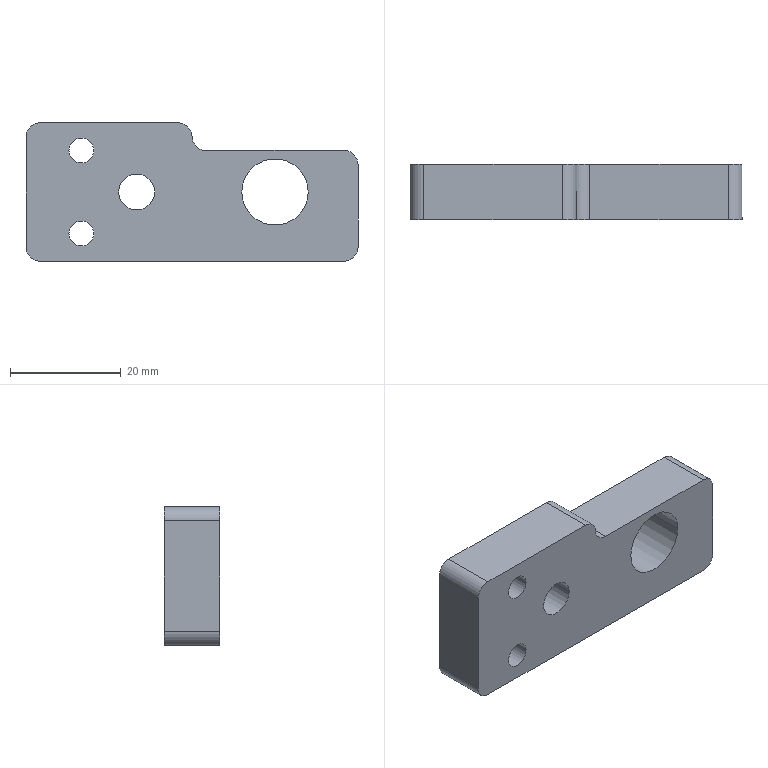Component | SolidWorks | GbgbGuidePlate120F8-1 | 1 solid | 27 faces | box 60 x 10 x 25 mm | volume 11349 mm3 | cylinder 18 | plane 9 | commonest cylinder face diameters 5 x6 8 x4 4.5 x4 12 x2 6.5 x2
STEP:
#1=COLOUR_RGB('',0.7922,0.8196,0.9333);
#2=FILL_AREA_STYLE_COLOUR('',#1);
#3=FILL_AREA_STYLE('',(#2));
#4=SURFACE_STYLE_FILL_AREA(#3);
#5=SURFACE_SIDE_STYLE('',(#4));
#6=SURFACE_STYLE_USAGE(.BOTH.,#5);
#7=PRESENTATION_STYLE_ASSIGNMENT((#6));
#8=CARTESIAN_POINT('',(1.632,15.466,17.234));
#9=VERTEX_POINT('',#8);
#10=CARTESIAN_POINT('',(1.947,15.466,17.234));
#11=VERTEX_POINT('',#10);
#12=CARTESIAN_POINT('',(1.789,15.466,17.234));
#13=DIRECTION('',(-0.,1.,0.));
#14=DIRECTION('',(1.,0.,0.));
#15=AXIS2_PLACEMENT_3D('',#12,#13,#14);
#16=CIRCLE('',#15,0.1575);
#17=EDGE_CURVE('',#9,#11,#16,.T.);
#18=ORIENTED_EDGE('',*,*,#17,.F.);
#19=CARTESIAN_POINT('',(1.632,15.647,17.234));
#20=VERTEX_POINT('',#19);
#21=CARTESIAN_POINT('',(1.632,15.647,17.234));
#22=DIRECTION('',(-0.,1.,0.));
#23=VECTOR('',#22,39.37);
#24=LINE('',#21,#23);
#25=EDGE_CURVE('',#9,#20,#24,.T.);
#26=ORIENTED_EDGE('',*,*,#25,.T.);
#27=CARTESIAN_POINT('',(1.947,15.647,17.234));
#28=VERTEX_POINT('',#27);
#29=CARTESIAN_POINT('',(1.789,15.647,17.234));
#30=DIRECTION('',(-0.,1.,0.));
#31=DIRECTION('',(1.,0.,0.));
#32=AXIS2_PLACEMENT_3D('',#29,#30,#31);
#33=CIRCLE('',#32,0.1575);
#34=EDGE_CURVE('',#20,#28,#33,.T.);
#35=ORIENTED_EDGE('',*,*,#34,.T.);
#36=CARTESIAN_POINT('',(1.947,15.647,17.234));
#37=DIRECTION('',(-0.,1.,0.));
#38=VECTOR('',#37,39.37);
#39=LINE('',#36,#38);
#40=EDGE_CURVE('',#11,#28,#39,.T.);
#41=ORIENTED_EDGE('',*,*,#40,.F.);
#42=EDGE_LOOP('',(#18,#26,#35,#41));
#43=FACE_OUTER_BOUND('',#42,.T.);
#44=CARTESIAN_POINT('',(1.789,15.647,17.234));
#45=DIRECTION('',(-0.,1.,0.));
#46=DIRECTION('',(1.,0.,0.));
#47=AXIS2_PLACEMENT_3D('',#44,#45,#46);
#48=CYLINDRICAL_SURFACE('',#47,0.1575);
#49=ADVANCED_FACE('',(#43),#48,.F.);
#50=CARTESIAN_POINT('',(1.701,15.254,17.234));
#51=VERTEX_POINT('',#50);
#52=CARTESIAN_POINT('',(1.878,15.254,17.234));
#53=VERTEX_POINT('',#52);
#54=CARTESIAN_POINT('',(1.789,15.254,17.234));
#55=DIRECTION('',(-0.,1.,0.));
#56=DIRECTION('',(1.,0.,0.));
#57=AXIS2_PLACEMENT_3D('',#54,#55,#56);
#58=CIRCLE('',#57,0.08858);
#59=EDGE_CURVE('',#51,#53,#58,.T.);
#60=ORIENTED_EDGE('',*,*,#59,.F.);
#61=CARTESIAN_POINT('',(1.701,15.466,17.234));
#62=VERTEX_POINT('',#61);
#63=CARTESIAN_POINT('',(1.701,15.647,17.234));
#64=DIRECTION('',(-0.,1.,0.));
#65=VECTOR('',#64,39.37);
#66=LINE('',#63,#65);
#67=EDGE_CURVE('',#51,#62,#66,.T.);
#68=ORIENTED_EDGE('',*,*,#67,.T.);
#69=CARTESIAN_POINT('',(1.878,15.466,17.234));
#70=VERTEX_POINT('',#69);
#71=CARTESIAN_POINT('',(1.789,15.466,17.234));
#72=DIRECTION('',(-0.,1.,0.));
#73=DIRECTION('',(1.,0.,0.));
#74=AXIS2_PLACEMENT_3D('',#71,#72,#73);
#75=CIRCLE('',#74,0.08858);
#76=EDGE_CURVE('',#62,#70,#75,.T.);
#77=ORIENTED_EDGE('',*,*,#76,.T.);
#78=CARTESIAN_POINT('',(1.878,15.647,17.234));
#79=DIRECTION('',(-0.,1.,0.));
#80=VECTOR('',#79,39.37);
#81=LINE('',#78,#80);
#82=EDGE_CURVE('',#53,#70,#81,.T.);
#83=ORIENTED_EDGE('',*,*,#82,.F.);
#84=EDGE_LOOP('',(#60,#68,#77,#83));
#85=FACE_OUTER_BOUND('',#84,.T.);
#86=CARTESIAN_POINT('',(1.789,15.647,17.234));
#87=DIRECTION('',(-0.,1.,0.));
#88=DIRECTION('',(1.,0.,0.));
#89=AXIS2_PLACEMENT_3D('',#86,#87,#88);
#90=CYLINDRICAL_SURFACE('',#89,0.08858);
#91=ADVANCED_FACE('',(#85),#90,.F.);
#92=CARTESIAN_POINT('',(1.632,15.466,16.643));
#93=VERTEX_POINT('',#92);
#94=CARTESIAN_POINT('',(1.947,15.466,16.643));
#95=VERTEX_POINT('',#94);
#96=CARTESIAN_POINT('',(1.789,15.466,16.643));
#97=DIRECTION('',(-0.,1.,0.));
#98=DIRECTION('',(1.,0.,0.));
#99=AXIS2_PLACEMENT_3D('',#96,#97,#98);
#100=CIRCLE('',#99,0.1575);
#101=EDGE_CURVE('',#93,#95,#100,.T.);
#102=ORIENTED_EDGE('',*,*,#101,.F.);
#103=CARTESIAN_POINT('',(1.632,15.647,16.643));
#104=VERTEX_POINT('',#103);
#105=CARTESIAN_POINT('',(1.632,15.647,16.643));
#106=DIRECTION('',(-0.,1.,0.));
#107=VECTOR('',#106,39.37);
#108=LINE('',#105,#107);
#109=EDGE_CURVE('',#93,#104,#108,.T.);
#110=ORIENTED_EDGE('',*,*,#109,.T.);
#111=CARTESIAN_POINT('',(1.947,15.647,16.643));
#112=VERTEX_POINT('',#111);
#113=CARTESIAN_POINT('',(1.789,15.647,16.643));
#114=DIRECTION('',(-0.,1.,0.));
#115=DIRECTION('',(1.,0.,0.));
#116=AXIS2_PLACEMENT_3D('',#113,#114,#115);
#117=CIRCLE('',#116,0.1575);
#118=EDGE_CURVE('',#104,#112,#117,.T.);
#119=ORIENTED_EDGE('',*,*,#118,.T.);
#120=CARTESIAN_POINT('',(1.947,15.647,16.643));
#121=DIRECTION('',(-0.,1.,0.));
#122=VECTOR('',#121,39.37);
#123=LINE('',#120,#122);
#124=EDGE_CURVE('',#95,#112,#123,.T.);
#125=ORIENTED_EDGE('',*,*,#124,.F.);
#126=EDGE_LOOP('',(#102,#110,#119,#125));
#127=FACE_OUTER_BOUND('',#126,.T.);
#128=CARTESIAN_POINT('',(1.789,15.647,16.643));
#129=DIRECTION('',(-0.,1.,0.));
#130=DIRECTION('',(1.,0.,0.));
#131=AXIS2_PLACEMENT_3D('',#128,#129,#130);
#132=CYLINDRICAL_SURFACE('',#131,0.1575);
#133=ADVANCED_FACE('',(#127),#132,.F.);
#134=CARTESIAN_POINT('',(1.701,15.254,16.643));
#135=VERTEX_POINT('',#134);
#136=CARTESIAN_POINT('',(1.878,15.254,16.643));
#137=VERTEX_POINT('',#136);
#138=CARTESIAN_POINT('',(1.789,15.254,16.643));
#139=DIRECTION('',(-0.,1.,0.));
#140=DIRECTION('',(1.,0.,0.));
#141=AXIS2_PLACEMENT_3D('',#138,#139,#140);
#142=CIRCLE('',#141,0.08858);
#143=EDGE_CURVE('',#135,#137,#142,.T.);
#144=ORIENTED_EDGE('',*,*,#143,.F.);
#145=CARTESIAN_POINT('',(1.701,15.466,16.643));
#146=VERTEX_POINT('',#145);
#147=CARTESIAN_POINT('',(1.701,15.647,16.643));
#148=DIRECTION('',(-0.,1.,0.));
#149=VECTOR('',#148,39.37);
#150=LINE('',#147,#149);
#151=EDGE_CURVE('',#135,#146,#150,.T.);
#152=ORIENTED_EDGE('',*,*,#151,.T.);
#153=CARTESIAN_POINT('',(1.878,15.466,16.643));
#154=VERTEX_POINT('',#153);
#155=CARTESIAN_POINT('',(1.789,15.466,16.643));
#156=DIRECTION('',(-0.,1.,0.));
#157=DIRECTION('',(1.,0.,0.));
#158=AXIS2_PLACEMENT_3D('',#155,#156,#157);
#159=CIRCLE('',#158,0.08858);
#160=EDGE_CURVE('',#146,#154,#159,.T.);
#161=ORIENTED_EDGE('',*,*,#160,.T.);
#162=CARTESIAN_POINT('',(1.878,15.647,16.643));
#163=DIRECTION('',(-0.,1.,0.));
#164=VECTOR('',#163,39.37);
#165=LINE('',#162,#164);
#166=EDGE_CURVE('',#137,#154,#165,.T.);
#167=ORIENTED_EDGE('',*,*,#166,.F.);
#168=EDGE_LOOP('',(#144,#152,#161,#167));
#169=FACE_OUTER_BOUND('',#168,.T.);
#170=CARTESIAN_POINT('',(1.789,15.647,16.643));
#171=DIRECTION('',(-0.,1.,0.));
#172=DIRECTION('',(1.,0.,0.));
#173=AXIS2_PLACEMENT_3D('',#170,#171,#172);
#174=CYLINDRICAL_SURFACE('',#173,0.08858);
#175=ADVANCED_FACE('',(#169),#174,.F.);
#176=CARTESIAN_POINT('',(2.931,15.254,16.938));
#177=VERTEX_POINT('',#176);
#178=CARTESIAN_POINT('',(3.403,15.254,16.938));
#179=VERTEX_POINT('',#178);
#180=CARTESIAN_POINT('',(3.167,15.254,16.938));
#181=DIRECTION('',(-0.,1.,0.));
#182=DIRECTION('',(1.,0.,0.));
#183=AXIS2_PLACEMENT_3D('',#180,#181,#182);
#184=CIRCLE('',#183,0.2362);
#185=EDGE_CURVE('',#177,#179,#184,.T.);
#186=ORIENTED_EDGE('',*,*,#185,.F.);
#187=CARTESIAN_POINT('',(2.931,15.647,16.938));
#188=VERTEX_POINT('',#187);
#189=CARTESIAN_POINT('',(2.931,15.254,16.938));
#190=DIRECTION('',(-0.,1.,0.));
#191=VECTOR('',#190,39.37);
#192=LINE('',#189,#191);
#193=EDGE_CURVE('',#177,#188,#192,.T.);
#194=ORIENTED_EDGE('',*,*,#193,.T.);
#195=CARTESIAN_POINT('',(3.403,15.647,16.938));
#196=VERTEX_POINT('',#195);
#197=CARTESIAN_POINT('',(3.167,15.647,16.938));
#198=DIRECTION('',(-0.,1.,0.));
#199=DIRECTION('',(1.,0.,0.));
#200=AXIS2_PLACEMENT_3D('',#197,#198,#199);
#201=CIRCLE('',#200,0.2362);
#202=EDGE_CURVE('',#188,#196,#201,.T.);
#203=ORIENTED_EDGE('',*,*,#202,.T.);
#204=CARTESIAN_POINT('',(3.403,15.254,16.938));
#205=DIRECTION('',(-0.,1.,0.));
#206=VECTOR('',#205,39.37);
#207=LINE('',#204,#206);
#208=EDGE_CURVE('',#179,#196,#207,.T.);
#209=ORIENTED_EDGE('',*,*,#208,.F.);
#210=EDGE_LOOP('',(#186,#194,#203,#209));
#211=FACE_OUTER_BOUND('',#210,.T.);
#212=CARTESIAN_POINT('',(3.167,15.254,16.938));
#213=DIRECTION('',(-0.,1.,0.));
#214=DIRECTION('',(1.,0.,0.));
#215=AXIS2_PLACEMENT_3D('',#212,#213,#214);
#216=CYLINDRICAL_SURFACE('',#215,0.2362);
#217=ADVANCED_FACE('',(#211),#216,.F.);
#218=CARTESIAN_POINT('',(2.055,15.254,16.938));
#219=VERTEX_POINT('',#218);
#220=CARTESIAN_POINT('',(2.311,15.254,16.938));
#221=VERTEX_POINT('',#220);
#222=CARTESIAN_POINT('',(2.183,15.254,16.938));
#223=DIRECTION('',(-0.,1.,0.));
#224=DIRECTION('',(1.,0.,0.));
#225=AXIS2_PLACEMENT_3D('',#222,#223,#224);
#226=CIRCLE('',#225,0.128);
#227=EDGE_CURVE('',#219,#221,#226,.T.);
#228=ORIENTED_EDGE('',*,*,#227,.F.);
#229=CARTESIAN_POINT('',(2.055,15.647,16.938));
#230=VERTEX_POINT('',#229);
#231=CARTESIAN_POINT('',(2.055,15.254,16.938));
#232=DIRECTION('',(-0.,1.,0.));
#233=VECTOR('',#232,39.37);
#234=LINE('',#231,#233);
#235=EDGE_CURVE('',#219,#230,#234,.T.);
#236=ORIENTED_EDGE('',*,*,#235,.T.);
#237=CARTESIAN_POINT('',(2.311,15.647,16.938));
#238=VERTEX_POINT('',#237);
#239=CARTESIAN_POINT('',(2.183,15.647,16.938));
#240=DIRECTION('',(-0.,1.,0.));
#241=DIRECTION('',(1.,0.,0.));
#242=AXIS2_PLACEMENT_3D('',#239,#240,#241);
#243=CIRCLE('',#242,0.128);
#244=EDGE_CURVE('',#230,#238,#243,.T.);
#245=ORIENTED_EDGE('',*,*,#244,.T.);
#246=CARTESIAN_POINT('',(2.311,15.254,16.938));
#247=DIRECTION('',(-0.,1.,0.));
#248=VECTOR('',#247,39.37);
#249=LINE('',#246,#248);
#250=EDGE_CURVE('',#221,#238,#249,.T.);
#251=ORIENTED_EDGE('',*,*,#250,.F.);
#252=EDGE_LOOP('',(#228,#236,#245,#251));
#253=FACE_OUTER_BOUND('',#252,.T.);
#254=CARTESIAN_POINT('',(2.183,15.254,16.938));
#255=DIRECTION('',(-0.,1.,0.));
#256=DIRECTION('',(1.,0.,0.));
#257=AXIS2_PLACEMENT_3D('',#254,#255,#256);
#258=CYLINDRICAL_SURFACE('',#257,0.128);
#259=ADVANCED_FACE('',(#253),#258,.F.);
#260=CARTESIAN_POINT('',(3.659,15.254,16.446));
#261=VERTEX_POINT('',#260);
#262=CARTESIAN_POINT('',(1.494,15.254,16.446));
#263=VERTEX_POINT('',#262);
#264=CARTESIAN_POINT('',(1.396,15.254,16.446));
#265=DIRECTION('',(-1.,-0.,0.));
#266=VECTOR('',#265,39.37);
#267=LINE('',#264,#266);
#268=EDGE_CURVE('',#261,#263,#267,.T.);
#269=ORIENTED_EDGE('',*,*,#268,.T.);
#270=CARTESIAN_POINT('',(1.494,15.647,16.446));
#271=VERTEX_POINT('',#270);
#272=CARTESIAN_POINT('',(1.494,15.647,16.446));
#273=DIRECTION('',(-0.,1.,0.));
#274=VECTOR('',#273,39.37);
#275=LINE('',#272,#274);
#276=EDGE_CURVE('',#263,#271,#275,.T.);
#277=ORIENTED_EDGE('',*,*,#276,.T.);
#278=CARTESIAN_POINT('',(3.659,15.647,16.446));
#279=VERTEX_POINT('',#278);
#280=CARTESIAN_POINT('',(1.396,15.647,16.446));
#281=DIRECTION('',(-1.,-0.,0.));
#282=VECTOR('',#281,39.37);
#283=LINE('',#280,#282);
#284=EDGE_CURVE('',#279,#271,#283,.T.);
#285=ORIENTED_EDGE('',*,*,#284,.F.);
#286=CARTESIAN_POINT('',(3.659,15.647,16.446));
#287=DIRECTION('',(0.,-1.,-0.));
#288=VECTOR('',#287,39.37);
#289=LINE('',#286,#288);
#290=EDGE_CURVE('',#279,#261,#289,.T.);
#291=ORIENTED_EDGE('',*,*,#290,.T.);
#292=EDGE_LOOP('',(#269,#277,#285,#291));
#293=FACE_OUTER_BOUND('',#292,.T.);
#294=CARTESIAN_POINT('',(1.396,15.647,16.446));
#295=DIRECTION('',(0.,-0.,1.));
#296=DIRECTION('',(1.,0.,-0.));
#297=AXIS2_PLACEMENT_3D('',#294,#295,#296);
#298=PLANE('',#297);
#299=ADVANCED_FACE('',(#293),#298,.F.);
#300=CARTESIAN_POINT('',(1.396,15.647,16.545));
#301=VERTEX_POINT('',#300);
#302=CARTESIAN_POINT('',(1.396,15.647,17.332));
#303=VERTEX_POINT('',#302);
#304=CARTESIAN_POINT('',(1.396,15.647,17.43));
#305=DIRECTION('',(0.,-0.,1.));
#306=VECTOR('',#305,39.37);
#307=LINE('',#304,#306);
#308=EDGE_CURVE('',#301,#303,#307,.T.);
#309=ORIENTED_EDGE('',*,*,#308,.F.);
#310=CARTESIAN_POINT('',(1.396,15.254,16.545));
#311=VERTEX_POINT('',#310);
#312=CARTESIAN_POINT('',(1.396,15.647,16.545));
#313=DIRECTION('',(0.,-1.,-0.));
#314=VECTOR('',#313,39.37);
#315=LINE('',#312,#314);
#316=EDGE_CURVE('',#301,#311,#315,.T.);
#317=ORIENTED_EDGE('',*,*,#316,.T.);
#318=CARTESIAN_POINT('',(1.396,15.254,17.332));
#319=VERTEX_POINT('',#318);
#320=CARTESIAN_POINT('',(1.396,15.254,17.43));
#321=DIRECTION('',(0.,-0.,1.));
#322=VECTOR('',#321,39.37);
#323=LINE('',#320,#322);
#324=EDGE_CURVE('',#311,#319,#323,.T.);
#325=ORIENTED_EDGE('',*,*,#324,.T.);
#326=CARTESIAN_POINT('',(1.396,15.647,17.332));
#327=DIRECTION('',(-0.,1.,0.));
#328=VECTOR('',#327,39.37);
#329=LINE('',#326,#328);
#330=EDGE_CURVE('',#319,#303,#329,.T.);
#331=ORIENTED_EDGE('',*,*,#330,.T.);
#332=EDGE_LOOP('',(#309,#317,#325,#331));
#333=FACE_OUTER_BOUND('',#332,.T.);
#334=CARTESIAN_POINT('',(1.396,15.647,17.43));
#335=DIRECTION('',(1.,0.,-0.));
#336=DIRECTION('',(-0.,0.,-1.));
#337=AXIS2_PLACEMENT_3D('',#334,#335,#336);
#338=PLANE('',#337);
#339=ADVANCED_FACE('',(#333),#338,.F.);
#340=CARTESIAN_POINT('',(1.494,15.647,17.43));
#341=VERTEX_POINT('',#340);
#342=CARTESIAN_POINT('',(2.478,15.647,17.43));
#343=VERTEX_POINT('',#342);
#344=CARTESIAN_POINT('',(1.396,15.647,17.43));
#345=DIRECTION('',(1.,0.,-0.));
#346=VECTOR('',#345,39.37);
#347=LINE('',#344,#346);
#348=EDGE_CURVE('',#341,#343,#347,.T.);
#349=ORIENTED_EDGE('',*,*,#348,.F.);
#350=CARTESIAN_POINT('',(1.494,15.254,17.43));
#351=VERTEX_POINT('',#350);
#352=CARTESIAN_POINT('',(1.494,15.647,17.43));
#353=DIRECTION('',(0.,-1.,-0.));
#354=VECTOR('',#353,39.37);
#355=LINE('',#352,#354);
#356=EDGE_CURVE('',#341,#351,#355,.T.);
#357=ORIENTED_EDGE('',*,*,#356,.T.);
#358=CARTESIAN_POINT('',(2.478,15.254,17.43));
#359=VERTEX_POINT('',#358);
#360=CARTESIAN_POINT('',(1.396,15.254,17.43));
#361=DIRECTION('',(1.,0.,-0.));
#362=VECTOR('',#361,39.37);
#363=LINE('',#360,#362);
#364=EDGE_CURVE('',#351,#359,#363,.T.);
#365=ORIENTED_EDGE('',*,*,#364,.T.);
#366=CARTESIAN_POINT('',(2.478,15.647,17.43));
#367=DIRECTION('',(-0.,1.,0.));
#368=VECTOR('',#367,39.37);
#369=LINE('',#366,#368);
#370=EDGE_CURVE('',#359,#343,#369,.T.);
#371=ORIENTED_EDGE('',*,*,#370,.T.);
#372=EDGE_LOOP('',(#349,#357,#365,#371));
#373=FACE_OUTER_BOUND('',#372,.T.);
#374=CARTESIAN_POINT('',(1.396,15.647,17.43));
#375=DIRECTION('',(-0.,0.,-1.));
#376=DIRECTION('',(-1.,-0.,0.));
#377=AXIS2_PLACEMENT_3D('',#374,#375,#376);
#378=PLANE('',#377);
#379=ADVANCED_FACE('',(#373),#378,.F.);
#380=CARTESIAN_POINT('',(3.758,15.254,17.135));
#381=VERTEX_POINT('',#380);
#382=CARTESIAN_POINT('',(3.758,15.254,16.545));
#383=VERTEX_POINT('',#382);
#384=CARTESIAN_POINT('',(3.758,15.254,17.43));
#385=DIRECTION('',(-0.,0.,-1.));
#386=VECTOR('',#385,39.37);
#387=LINE('',#384,#386);
#388=EDGE_CURVE('',#381,#383,#387,.T.);
#389=ORIENTED_EDGE('',*,*,#388,.T.);
#390=CARTESIAN_POINT('',(3.758,15.647,16.545));
#391=VERTEX_POINT('',#390);
#392=CARTESIAN_POINT('',(3.758,15.647,16.545));
#393=DIRECTION('',(-0.,1.,0.));
#394=VECTOR('',#393,39.37);
#395=LINE('',#392,#394);
#396=EDGE_CURVE('',#383,#391,#395,.T.);
#397=ORIENTED_EDGE('',*,*,#396,.T.);
#398=CARTESIAN_POINT('',(3.758,15.647,17.135));
#399=VERTEX_POINT('',#398);
#400=CARTESIAN_POINT('',(3.758,15.647,17.43));
#401=DIRECTION('',(-0.,0.,-1.));
#402=VECTOR('',#401,39.37);
#403=LINE('',#400,#402);
#404=EDGE_CURVE('',#399,#391,#403,.T.);
#405=ORIENTED_EDGE('',*,*,#404,.F.);
#406=CARTESIAN_POINT('',(3.758,15.647,17.135));
#407=DIRECTION('',(0.,-1.,-0.));
#408=VECTOR('',#407,39.37);
#409=LINE('',#406,#408);
#410=EDGE_CURVE('',#399,#381,#409,.T.);
#411=ORIENTED_EDGE('',*,*,#410,.T.);
#412=EDGE_LOOP('',(#389,#397,#405,#411));
#413=FACE_OUTER_BOUND('',#412,.T.);
#414=CARTESIAN_POINT('',(3.758,15.647,17.43));
#415=DIRECTION('',(-1.,-0.,0.));
#416=DIRECTION('',(0.,-0.,1.));
#417=AXIS2_PLACEMENT_3D('',#414,#415,#416);
#418=PLANE('',#417);
#419=ADVANCED_FACE('',(#413),#418,.F.);
#420=CARTESIAN_POINT('',(1.789,15.647,17.234));
#421=DIRECTION('',(-0.,1.,0.));
#422=DIRECTION('',(1.,0.,0.));
#423=AXIS2_PLACEMENT_3D('',#420,#421,#422);
#424=CIRCLE('',#423,0.1575);
#425=EDGE_CURVE('',#28,#20,#424,.T.);
#426=ORIENTED_EDGE('',*,*,#425,.F.);
#427=ORIENTED_EDGE('',*,*,#34,.F.);
#428=EDGE_LOOP('',(#426,#427));
#429=FACE_BOUND('',#428,.T.);
#430=CARTESIAN_POINT('',(1.789,15.647,16.643));
#431=DIRECTION('',(-0.,1.,0.));
#432=DIRECTION('',(1.,0.,0.));
#433=AXIS2_PLACEMENT_3D('',#430,#431,#432);
#434=CIRCLE('',#433,0.1575);
#435=EDGE_CURVE('',#112,#104,#434,.T.);
#436=ORIENTED_EDGE('',*,*,#435,.F.);
#437=ORIENTED_EDGE('',*,*,#118,.F.);
#438=EDGE_LOOP('',(#436,#437));
#439=FACE_BOUND('',#438,.T.);
#440=ORIENTED_EDGE('',*,*,#284,.T.);
#441=CARTESIAN_POINT('',(1.494,15.647,16.545));
#442=DIRECTION('',(-0.,1.,0.));
#443=DIRECTION('',(1.,0.,0.));
#444=AXIS2_PLACEMENT_3D('',#441,#442,#443);
#445=CIRCLE('',#444,0.09843);
#446=EDGE_CURVE('',#271,#301,#445,.T.);
#447=ORIENTED_EDGE('',*,*,#446,.T.);
#448=ORIENTED_EDGE('',*,*,#308,.T.);
#449=CARTESIAN_POINT('',(1.494,15.647,17.332));
#450=DIRECTION('',(-0.,1.,0.));
#451=DIRECTION('',(1.,0.,0.));
#452=AXIS2_PLACEMENT_3D('',#449,#450,#451);
#453=CIRCLE('',#452,0.09843);
#454=EDGE_CURVE('',#303,#341,#453,.T.);
#455=ORIENTED_EDGE('',*,*,#454,.T.);
#456=ORIENTED_EDGE('',*,*,#348,.T.);
#457=CARTESIAN_POINT('',(2.577,15.647,17.332));
#458=VERTEX_POINT('',#457);
#459=CARTESIAN_POINT('',(2.478,15.647,17.332));
#460=DIRECTION('',(-0.,1.,0.));
#461=DIRECTION('',(1.,0.,0.));
#462=AXIS2_PLACEMENT_3D('',#459,#460,#461);
#463=CIRCLE('',#462,0.09843);
#464=EDGE_CURVE('',#343,#458,#463,.T.);
#465=ORIENTED_EDGE('',*,*,#464,.T.);
#466=CARTESIAN_POINT('',(2.675,15.647,17.234));
#467=VERTEX_POINT('',#466);
#468=CARTESIAN_POINT('',(2.675,15.647,17.332));
#469=DIRECTION('',(0.,-1.,-0.));
#470=DIRECTION('',(1.,0.,0.));
#471=AXIS2_PLACEMENT_3D('',#468,#469,#470);
#472=CIRCLE('',#471,0.09843);
#473=EDGE_CURVE('',#458,#467,#472,.T.);
#474=ORIENTED_EDGE('',*,*,#473,.T.);
#475=CARTESIAN_POINT('',(3.659,15.647,17.234));
#476=VERTEX_POINT('',#475);
#477=CARTESIAN_POINT('',(2.577,15.647,17.234));
#478=DIRECTION('',(-1.,-0.,0.));
#479=VECTOR('',#478,39.37);
#480=LINE('',#477,#479);
#481=EDGE_CURVE('',#476,#467,#480,.T.);
#482=ORIENTED_EDGE('',*,*,#481,.F.);
#483=CARTESIAN_POINT('',(3.659,15.647,17.135));
#484=DIRECTION('',(-0.,1.,0.));
#485=DIRECTION('',(1.,0.,0.));
#486=AXIS2_PLACEMENT_3D('',#483,#484,#485);
#487=CIRCLE('',#486,0.09843);
#488=EDGE_CURVE('',#476,#399,#487,.T.);
#489=ORIENTED_EDGE('',*,*,#488,.T.);
#490=ORIENTED_EDGE('',*,*,#404,.T.);
#491=CARTESIAN_POINT('',(3.659,15.647,16.545));
#492=DIRECTION('',(-0.,1.,0.));
#493=DIRECTION('',(1.,0.,0.));
#494=AXIS2_PLACEMENT_3D('',#491,#492,#493);
#495=CIRCLE('',#494,0.09843);
#496=EDGE_CURVE('',#391,#279,#495,.T.);
#497=ORIENTED_EDGE('',*,*,#496,.T.);
#498=EDGE_LOOP('',(#440,#447,#448,#455,#456,#465,#474,#482,#489,#490,#497));
#499=FACE_OUTER_BOUND('',#498,.T.);
#500=CARTESIAN_POINT('',(3.167,15.647,16.938));
#501=DIRECTION('',(-0.,1.,0.));
#502=DIRECTION('',(1.,0.,0.));
#503=AXIS2_PLACEMENT_3D('',#500,#501,#502);
#504=CIRCLE('',#503,0.2362);
#505=EDGE_CURVE('',#196,#188,#504,.T.);
#506=ORIENTED_EDGE('',*,*,#505,.F.);
#507=ORIENTED_EDGE('',*,*,#202,.F.);
#508=EDGE_LOOP('',(#506,#507));
#509=FACE_BOUND('',#508,.T.);
#510=CARTESIAN_POINT('',(2.183,15.647,16.938));
#511=DIRECTION('',(-0.,1.,0.));
#512=DIRECTION('',(1.,0.,0.));
#513=AXIS2_PLACEMENT_3D('',#510,#511,#512);
#514=CIRCLE('',#513,0.128);
#515=EDGE_CURVE('',#238,#230,#514,.T.);
#516=ORIENTED_EDGE('',*,*,#515,.F.);
#517=ORIENTED_EDGE('',*,*,#244,.F.);
#518=EDGE_LOOP('',(#516,#517));
#519=FACE_BOUND('',#518,.T.);
#520=CARTESIAN_POINT('',(2.577,15.647,16.938));
#521=DIRECTION('',(-0.,1.,0.));
#522=DIRECTION('',(1.,0.,-0.));
#523=AXIS2_PLACEMENT_3D('',#520,#521,#522);
#524=PLANE('',#523);
#525=ADVANCED_FACE('',(#429,#439,#499,#509,#519),#524,.T.);
#526=CARTESIAN_POINT('',(1.789,15.254,17.234));
#527=DIRECTION('',(-0.,1.,0.));
#528=DIRECTION('',(1.,0.,0.));
#529=AXIS2_PLACEMENT_3D('',#526,#527,#528);
#530=CIRCLE('',#529,0.08858);
#531=EDGE_CURVE('',#53,#51,#530,.T.);
#532=ORIENTED_EDGE('',*,*,#531,.T.);
#533=ORIENTED_EDGE('',*,*,#59,.T.);
#534=EDGE_LOOP('',(#532,#533));
#535=FACE_BOUND('',#534,.T.);
#536=CARTESIAN_POINT('',(1.789,15.254,16.643));
#537=DIRECTION('',(-0.,1.,0.));
#538=DIRECTION('',(1.,0.,0.));
#539=AXIS2_PLACEMENT_3D('',#536,#537,#538);
#540=CIRCLE('',#539,0.08858);
#541=EDGE_CURVE('',#137,#135,#540,.T.);
#542=ORIENTED_EDGE('',*,*,#541,.T.);
#543=ORIENTED_EDGE('',*,*,#143,.T.);
#544=EDGE_LOOP('',(#542,#543));
#545=FACE_BOUND('',#544,.T.);
#546=CARTESIAN_POINT('',(3.167,15.254,16.938));
#547=DIRECTION('',(-0.,1.,0.));
#548=DIRECTION('',(1.,0.,0.));
#549=AXIS2_PLACEMENT_3D('',#546,#547,#548);
#550=CIRCLE('',#549,0.2362);
#551=EDGE_CURVE('',#179,#177,#550,.T.);
#552=ORIENTED_EDGE('',*,*,#551,.T.);
#553=ORIENTED_EDGE('',*,*,#185,.T.);
#554=EDGE_LOOP('',(#552,#553));
#555=FACE_BOUND('',#554,.T.);
#556=CARTESIAN_POINT('',(2.183,15.254,16.938));
#557=DIRECTION('',(-0.,1.,0.));
#558=DIRECTION('',(1.,0.,0.));
#559=AXIS2_PLACEMENT_3D('',#556,#557,#558);
#560=CIRCLE('',#559,0.128);
#561=EDGE_CURVE('',#221,#219,#560,.T.);
#562=ORIENTED_EDGE('',*,*,#561,.T.);
#563=ORIENTED_EDGE('',*,*,#227,.T.);
#564=EDGE_LOOP('',(#562,#563));
#565=FACE_BOUND('',#564,.T.);
#566=ORIENTED_EDGE('',*,*,#324,.F.);
#567=CARTESIAN_POINT('',(1.494,15.254,16.545));
#568=DIRECTION('',(0.,-1.,-0.));
#569=DIRECTION('',(1.,0.,0.));
#570=AXIS2_PLACEMENT_3D('',#567,#568,#569);
#571=CIRCLE('',#570,0.09843);
#572=EDGE_CURVE('',#311,#263,#571,.T.);
#573=ORIENTED_EDGE('',*,*,#572,.T.);
#574=ORIENTED_EDGE('',*,*,#268,.F.);
#575=CARTESIAN_POINT('',(3.659,15.254,16.545));
#576=DIRECTION('',(0.,-1.,-0.));
#577=DIRECTION('',(1.,0.,0.));
#578=AXIS2_PLACEMENT_3D('',#575,#576,#577);
#579=CIRCLE('',#578,0.09843);
#580=EDGE_CURVE('',#261,#383,#579,.T.);
#581=ORIENTED_EDGE('',*,*,#580,.T.);
#582=ORIENTED_EDGE('',*,*,#388,.F.);
#583=CARTESIAN_POINT('',(3.659,15.254,17.234));
#584=VERTEX_POINT('',#583);
#585=CARTESIAN_POINT('',(3.659,15.254,17.135));
#586=DIRECTION('',(0.,-1.,-0.));
#587=DIRECTION('',(1.,0.,0.));
#588=AXIS2_PLACEMENT_3D('',#585,#586,#587);
#589=CIRCLE('',#588,0.09843);
#590=EDGE_CURVE('',#381,#584,#589,.T.);
#591=ORIENTED_EDGE('',*,*,#590,.T.);
#592=CARTESIAN_POINT('',(2.675,15.254,17.234));
#593=VERTEX_POINT('',#592);
#594=CARTESIAN_POINT('',(2.577,15.254,17.234));
#595=DIRECTION('',(-1.,-0.,0.));
#596=VECTOR('',#595,39.37);
#597=LINE('',#594,#596);
#598=EDGE_CURVE('',#584,#593,#597,.T.);
#599=ORIENTED_EDGE('',*,*,#598,.T.);
#600=CARTESIAN_POINT('',(2.577,15.254,17.332));
#601=VERTEX_POINT('',#600);
#602=CARTESIAN_POINT('',(2.675,15.254,17.332));
#603=DIRECTION('',(-0.,1.,0.));
#604=DIRECTION('',(1.,0.,0.));
#605=AXIS2_PLACEMENT_3D('',#602,#603,#604);
#606=CIRCLE('',#605,0.09843);
#607=EDGE_CURVE('',#593,#601,#606,.T.);
#608=ORIENTED_EDGE('',*,*,#607,.T.);
#609=CARTESIAN_POINT('',(2.478,15.254,17.332));
#610=DIRECTION('',(0.,-1.,-0.));
#611=DIRECTION('',(1.,0.,0.));
#612=AXIS2_PLACEMENT_3D('',#609,#610,#611);
#613=CIRCLE('',#612,0.09843);
#614=EDGE_CURVE('',#601,#359,#613,.T.);
#615=ORIENTED_EDGE('',*,*,#614,.T.);
#616=ORIENTED_EDGE('',*,*,#364,.F.);
#617=CARTESIAN_POINT('',(1.494,15.254,17.332));
#618=DIRECTION('',(0.,-1.,-0.));
#619=DIRECTION('',(1.,0.,0.));
#620=AXIS2_PLACEMENT_3D('',#617,#618,#619);
#621=CIRCLE('',#620,0.09843);
#622=EDGE_CURVE('',#351,#319,#621,.T.);
#623=ORIENTED_EDGE('',*,*,#622,.T.);
#624=EDGE_LOOP('',(#566,#573,#574,#581,#582,#591,#599,#608,#615,#616,#623));
#625=FACE_OUTER_BOUND('',#624,.T.);
#626=CARTESIAN_POINT('',(2.577,15.254,16.938));
#627=DIRECTION('',(-0.,1.,0.));
#628=DIRECTION('',(1.,0.,-0.));
#629=AXIS2_PLACEMENT_3D('',#626,#627,#628);
#630=PLANE('',#629);
#631=ADVANCED_FACE('',(#535,#545,#555,#565,#625),#630,.F.);
#632=ORIENTED_EDGE('',*,*,#235,.F.);
#633=ORIENTED_EDGE('',*,*,#561,.F.);
#634=ORIENTED_EDGE('',*,*,#250,.T.);
#635=ORIENTED_EDGE('',*,*,#515,.T.);
#636=EDGE_LOOP('',(#632,#633,#634,#635));
#637=FACE_OUTER_BOUND('',#636,.T.);
#638=CARTESIAN_POINT('',(2.183,15.254,16.938));
#639=DIRECTION('',(-0.,1.,0.));
#640=DIRECTION('',(1.,0.,0.));
#641=AXIS2_PLACEMENT_3D('',#638,#639,#640);
#642=CYLINDRICAL_SURFACE('',#641,0.128);
#643=ADVANCED_FACE('',(#637),#642,.F.);
#644=ORIENTED_EDGE('',*,*,#193,.F.);
#645=ORIENTED_EDGE('',*,*,#551,.F.);
#646=ORIENTED_EDGE('',*,*,#208,.T.);
#647=ORIENTED_EDGE('',*,*,#505,.T.);
#648=EDGE_LOOP('',(#644,#645,#646,#647));
#649=FACE_OUTER_BOUND('',#648,.T.);
#650=CARTESIAN_POINT('',(3.167,15.254,16.938));
#651=DIRECTION('',(-0.,1.,0.));
#652=DIRECTION('',(1.,0.,0.));
#653=AXIS2_PLACEMENT_3D('',#650,#651,#652);
#654=CYLINDRICAL_SURFACE('',#653,0.2362);
#655=ADVANCED_FACE('',(#649),#654,.F.);
#656=ORIENTED_EDGE('',*,*,#598,.F.);
#657=CARTESIAN_POINT('',(3.659,15.254,17.234));
#658=DIRECTION('',(-0.,1.,0.));
#659=VECTOR('',#658,39.37);
#660=LINE('',#657,#659);
#661=EDGE_CURVE('',#584,#476,#660,.T.);
#662=ORIENTED_EDGE('',*,*,#661,.T.);
#663=ORIENTED_EDGE('',*,*,#481,.T.);
#664=CARTESIAN_POINT('',(2.675,15.254,17.234));
#665=DIRECTION('',(0.,-1.,-0.));
#666=VECTOR('',#665,39.37);
#667=LINE('',#664,#666);
#668=EDGE_CURVE('',#467,#593,#667,.T.);
#669=ORIENTED_EDGE('',*,*,#668,.T.);
#670=EDGE_LOOP('',(#656,#662,#663,#669));
#671=FACE_OUTER_BOUND('',#670,.T.);
#672=CARTESIAN_POINT('',(2.577,15.254,17.234));
#673=DIRECTION('',(-0.,0.,-1.));
#674=DIRECTION('',(-1.,-0.,0.));
#675=AXIS2_PLACEMENT_3D('',#672,#673,#674);
#676=PLANE('',#675);
#677=ADVANCED_FACE('',(#671),#676,.F.);
#678=ORIENTED_EDGE('',*,*,#151,.F.);
#679=ORIENTED_EDGE('',*,*,#541,.F.);
#680=ORIENTED_EDGE('',*,*,#166,.T.);
#681=CARTESIAN_POINT('',(1.789,15.466,16.643));
#682=DIRECTION('',(-0.,1.,0.));
#683=DIRECTION('',(1.,0.,0.));
#684=AXIS2_PLACEMENT_3D('',#681,#682,#683);
#685=CIRCLE('',#684,0.08858);
#686=EDGE_CURVE('',#154,#146,#685,.T.);
#687=ORIENTED_EDGE('',*,*,#686,.T.);
#688=EDGE_LOOP('',(#678,#679,#680,#687));
#689=FACE_OUTER_BOUND('',#688,.T.);
#690=CARTESIAN_POINT('',(1.789,15.647,16.643));
#691=DIRECTION('',(-0.,1.,0.));
#692=DIRECTION('',(1.,0.,0.));
#693=AXIS2_PLACEMENT_3D('',#690,#691,#692);
#694=CYLINDRICAL_SURFACE('',#693,0.08858);
#695=ADVANCED_FACE('',(#689),#694,.F.);
#696=ORIENTED_EDGE('',*,*,#686,.F.);
#697=ORIENTED_EDGE('',*,*,#160,.F.);
#698=EDGE_LOOP('',(#696,#697));
#699=FACE_BOUND('',#698,.T.);
#700=CARTESIAN_POINT('',(1.789,15.466,16.643));
#701=DIRECTION('',(-0.,1.,0.));
#702=DIRECTION('',(1.,0.,0.));
#703=AXIS2_PLACEMENT_3D('',#700,#701,#702);
#704=CIRCLE('',#703,0.1575);
#705=EDGE_CURVE('',#95,#93,#704,.T.);
#706=ORIENTED_EDGE('',*,*,#705,.T.);
#707=ORIENTED_EDGE('',*,*,#101,.T.);
#708=EDGE_LOOP('',(#706,#707));
#709=FACE_OUTER_BOUND('',#708,.T.);
#710=CARTESIAN_POINT('',(1.789,15.466,16.554));
#711=DIRECTION('',(0.,-1.,-0.));
#712=DIRECTION('',(-1.,-0.,0.));
#713=AXIS2_PLACEMENT_3D('',#710,#711,#712);
#714=PLANE('',#713);
#715=ADVANCED_FACE('',(#699,#709),#714,.F.);
#716=ORIENTED_EDGE('',*,*,#109,.F.);
#717=ORIENTED_EDGE('',*,*,#705,.F.);
#718=ORIENTED_EDGE('',*,*,#124,.T.);
#719=ORIENTED_EDGE('',*,*,#435,.T.);
#720=EDGE_LOOP('',(#716,#717,#718,#719));
#721=FACE_OUTER_BOUND('',#720,.T.);
#722=CARTESIAN_POINT('',(1.789,15.647,16.643));
#723=DIRECTION('',(-0.,1.,0.));
#724=DIRECTION('',(1.,0.,0.));
#725=AXIS2_PLACEMENT_3D('',#722,#723,#724);
#726=CYLINDRICAL_SURFACE('',#725,0.1575);
#727=ADVANCED_FACE('',(#721),#726,.F.);
#728=ORIENTED_EDGE('',*,*,#67,.F.);
#729=ORIENTED_EDGE('',*,*,#531,.F.);
#730=ORIENTED_EDGE('',*,*,#82,.T.);
#731=CARTESIAN_POINT('',(1.789,15.466,17.234));
#732=DIRECTION('',(-0.,1.,0.));
#733=DIRECTION('',(1.,0.,0.));
#734=AXIS2_PLACEMENT_3D('',#731,#732,#733);
#735=CIRCLE('',#734,0.08858);
#736=EDGE_CURVE('',#70,#62,#735,.T.);
#737=ORIENTED_EDGE('',*,*,#736,.T.);
#738=EDGE_LOOP('',(#728,#729,#730,#737));
#739=FACE_OUTER_BOUND('',#738,.T.);
#740=CARTESIAN_POINT('',(1.789,15.647,17.234));
#741=DIRECTION('',(-0.,1.,0.));
#742=DIRECTION('',(1.,0.,0.));
#743=AXIS2_PLACEMENT_3D('',#740,#741,#742);
#744=CYLINDRICAL_SURFACE('',#743,0.08858);
#745=ADVANCED_FACE('',(#739),#744,.F.);
#746=ORIENTED_EDGE('',*,*,#736,.F.);
#747=ORIENTED_EDGE('',*,*,#76,.F.);
#748=EDGE_LOOP('',(#746,#747));
#749=FACE_BOUND('',#748,.T.);
#750=CARTESIAN_POINT('',(1.789,15.466,17.234));
#751=DIRECTION('',(-0.,1.,0.));
#752=DIRECTION('',(1.,0.,0.));
#753=AXIS2_PLACEMENT_3D('',#750,#751,#752);
#754=CIRCLE('',#753,0.1575);
#755=EDGE_CURVE('',#11,#9,#754,.T.);
#756=ORIENTED_EDGE('',*,*,#755,.T.);
#757=ORIENTED_EDGE('',*,*,#17,.T.);
#758=EDGE_LOOP('',(#756,#757));
#759=FACE_OUTER_BOUND('',#758,.T.);
#760=CARTESIAN_POINT('',(1.789,15.466,17.145));
#761=DIRECTION('',(0.,-1.,-0.));
#762=DIRECTION('',(-1.,-0.,0.));
#763=AXIS2_PLACEMENT_3D('',#760,#761,#762);
#764=PLANE('',#763);
#765=ADVANCED_FACE('',(#749,#759),#764,.F.);
#766=ORIENTED_EDGE('',*,*,#25,.F.);
#767=ORIENTED_EDGE('',*,*,#755,.F.);
#768=ORIENTED_EDGE('',*,*,#40,.T.);
#769=ORIENTED_EDGE('',*,*,#425,.T.);
#770=EDGE_LOOP('',(#766,#767,#768,#769));
#771=FACE_OUTER_BOUND('',#770,.T.);
#772=CARTESIAN_POINT('',(1.789,15.647,17.234));
#773=DIRECTION('',(-0.,1.,0.));
#774=DIRECTION('',(1.,0.,0.));
#775=AXIS2_PLACEMENT_3D('',#772,#773,#774);
#776=CYLINDRICAL_SURFACE('',#775,0.1575);
#777=ADVANCED_FACE('',(#771),#776,.F.);
#778=ORIENTED_EDGE('',*,*,#446,.F.);
#779=ORIENTED_EDGE('',*,*,#276,.F.);
#780=ORIENTED_EDGE('',*,*,#572,.F.);
#781=ORIENTED_EDGE('',*,*,#316,.F.);
#782=EDGE_LOOP('',(#778,#779,#780,#781));
#783=FACE_OUTER_BOUND('',#782,.T.);
#784=CARTESIAN_POINT('',(1.494,15.647,16.545));
#785=DIRECTION('',(0.,-1.,-0.));
#786=DIRECTION('',(-1.,-0.,0.));
#787=AXIS2_PLACEMENT_3D('',#784,#785,#786);
#788=CYLINDRICAL_SURFACE('',#787,0.09843);
#789=ADVANCED_FACE('',(#783),#788,.T.);
#790=ORIENTED_EDGE('',*,*,#454,.F.);
#791=ORIENTED_EDGE('',*,*,#330,.F.);
#792=ORIENTED_EDGE('',*,*,#622,.F.);
#793=ORIENTED_EDGE('',*,*,#356,.F.);
#794=EDGE_LOOP('',(#790,#791,#792,#793));
#795=FACE_OUTER_BOUND('',#794,.T.);
#796=CARTESIAN_POINT('',(1.494,15.647,17.332));
#797=DIRECTION('',(0.,-1.,-0.));
#798=DIRECTION('',(-1.,-0.,0.));
#799=AXIS2_PLACEMENT_3D('',#796,#797,#798);
#800=CYLINDRICAL_SURFACE('',#799,0.09843);
#801=ADVANCED_FACE('',(#795),#800,.T.);
#802=CARTESIAN_POINT('',(2.577,15.647,17.332));
#803=DIRECTION('',(-0.,1.,0.));
#804=VECTOR('',#803,39.37);
#805=LINE('',#802,#804);
#806=EDGE_CURVE('',#601,#458,#805,.T.);
#807=ORIENTED_EDGE('',*,*,#806,.F.);
#808=ORIENTED_EDGE('',*,*,#607,.F.);
#809=ORIENTED_EDGE('',*,*,#668,.F.);
#810=ORIENTED_EDGE('',*,*,#473,.F.);
#811=EDGE_LOOP('',(#807,#808,#809,#810));
#812=FACE_OUTER_BOUND('',#811,.T.);
#813=CARTESIAN_POINT('',(2.675,15.254,17.332));
#814=DIRECTION('',(0.,-1.,-0.));
#815=DIRECTION('',(-1.,-0.,0.));
#816=AXIS2_PLACEMENT_3D('',#813,#814,#815);
#817=CYLINDRICAL_SURFACE('',#816,0.09843);
#818=ADVANCED_FACE('',(#812),#817,.F.);
#819=ORIENTED_EDGE('',*,*,#614,.F.);
#820=ORIENTED_EDGE('',*,*,#806,.T.);
#821=ORIENTED_EDGE('',*,*,#464,.F.);
#822=ORIENTED_EDGE('',*,*,#370,.F.);
#823=EDGE_LOOP('',(#819,#820,#821,#822));
#824=FACE_OUTER_BOUND('',#823,.T.);
#825=CARTESIAN_POINT('',(2.478,15.647,17.332));
#826=DIRECTION('',(-0.,1.,0.));
#827=DIRECTION('',(1.,0.,0.));
#828=AXIS2_PLACEMENT_3D('',#825,#826,#827);
#829=CYLINDRICAL_SURFACE('',#828,0.09843);
#830=ADVANCED_FACE('',(#824),#829,.T.);
#831=ORIENTED_EDGE('',*,*,#496,.F.);
#832=ORIENTED_EDGE('',*,*,#396,.F.);
#833=ORIENTED_EDGE('',*,*,#580,.F.);
#834=ORIENTED_EDGE('',*,*,#290,.F.);
#835=EDGE_LOOP('',(#831,#832,#833,#834));
#836=FACE_OUTER_BOUND('',#835,.T.);
#837=CARTESIAN_POINT('',(3.659,15.647,16.545));
#838=DIRECTION('',(0.,-1.,-0.));
#839=DIRECTION('',(-1.,-0.,0.));
#840=AXIS2_PLACEMENT_3D('',#837,#838,#839);
#841=CYLINDRICAL_SURFACE('',#840,0.09843);
#842=ADVANCED_FACE('',(#836),#841,.T.);
#843=ORIENTED_EDGE('',*,*,#590,.F.);
#844=ORIENTED_EDGE('',*,*,#410,.F.);
#845=ORIENTED_EDGE('',*,*,#488,.F.);
#846=ORIENTED_EDGE('',*,*,#661,.F.);
#847=EDGE_LOOP('',(#843,#844,#845,#846));
#848=FACE_OUTER_BOUND('',#847,.T.);
#849=CARTESIAN_POINT('',(3.659,15.254,17.135));
#850=DIRECTION('',(-0.,1.,0.));
#851=DIRECTION('',(1.,0.,0.));
#852=AXIS2_PLACEMENT_3D('',#849,#850,#851);
#853=CYLINDRICAL_SURFACE('',#852,0.09843);
#854=ADVANCED_FACE('',(#848),#853,.T.);
#855=CLOSED_SHELL('',(#49,#91,#133,#175,#217,#259,#299,#339,#379,#419,#525,#631,#643,#655,#677,#695,#715,#727,#745,#765,#777,#789,#801,#818,#830,#842,#854));
#856=MANIFOLD_SOLID_BREP('',#855);
#857=STYLED_ITEM('',(#7),#856);
#858=(LENGTH_UNIT()NAMED_UNIT(*)SI_UNIT($,.METRE.));
#859=LENGTH_MEASURE_WITH_UNIT(LENGTH_MEASURE(0.0254),#858);
#860=DIMENSIONAL_EXPONENTS(1.,0.,0.,0.,0.,0.,0.);
#861=(CONVERSION_BASED_UNIT('',#859)LENGTH_UNIT()NAMED_UNIT(#860));
#862=UNCERTAINTY_MEASURE_WITH_UNIT(LENGTH_MEASURE(0.00001),#861,'','');
#863=(NAMED_UNIT(*)PLANE_ANGLE_UNIT()SI_UNIT($,.RADIAN.));
#864=(NAMED_UNIT(*)SI_UNIT($,.STERADIAN.)SOLID_ANGLE_UNIT());
#865=(GEOMETRIC_REPRESENTATION_CONTEXT(3)GLOBAL_UNCERTAINTY_ASSIGNED_CONTEXT((#862))GLOBAL_UNIT_ASSIGNED_CONTEXT((#861,#863,#864))REPRESENTATION_CONTEXT('',''));
#866=MECHANICAL_DESIGN_GEOMETRIC_PRESENTATION_REPRESENTATION('',(#857),#865);
#867=CARTESIAN_POINT('',(0.,0.,0.));
#868=DIRECTION('',(0.,0.,1.));
#869=DIRECTION('',(1.,0.,0.));
#870=AXIS2_PLACEMENT_3D('',#867,#868,#869);
#871=(LENGTH_UNIT()NAMED_UNIT(*)SI_UNIT($,.METRE.));
#872=LENGTH_MEASURE_WITH_UNIT(LENGTH_MEASURE(0.0254),#871);
#873=DIMENSIONAL_EXPONENTS(1.,0.,0.,0.,0.,0.,0.);
#874=(CONVERSION_BASED_UNIT('',#872)LENGTH_UNIT()NAMED_UNIT(#873));
#875=UNCERTAINTY_MEASURE_WITH_UNIT(LENGTH_MEASURE(0.00001),#874,'','');
#876=(NAMED_UNIT(*)PLANE_ANGLE_UNIT()SI_UNIT($,.RADIAN.));
#877=(NAMED_UNIT(*)SI_UNIT($,.STERADIAN.)SOLID_ANGLE_UNIT());
#878=(GEOMETRIC_REPRESENTATION_CONTEXT(3)GLOBAL_UNCERTAINTY_ASSIGNED_CONTEXT((#875))GLOBAL_UNIT_ASSIGNED_CONTEXT((#874,#876,#877))REPRESENTATION_CONTEXT('',''));
#879=ADVANCED_BREP_SHAPE_REPRESENTATION('',(#856,#870),#878);
#880=PRESENTATION_LAYER_ASSIGNMENT('','',(#857));